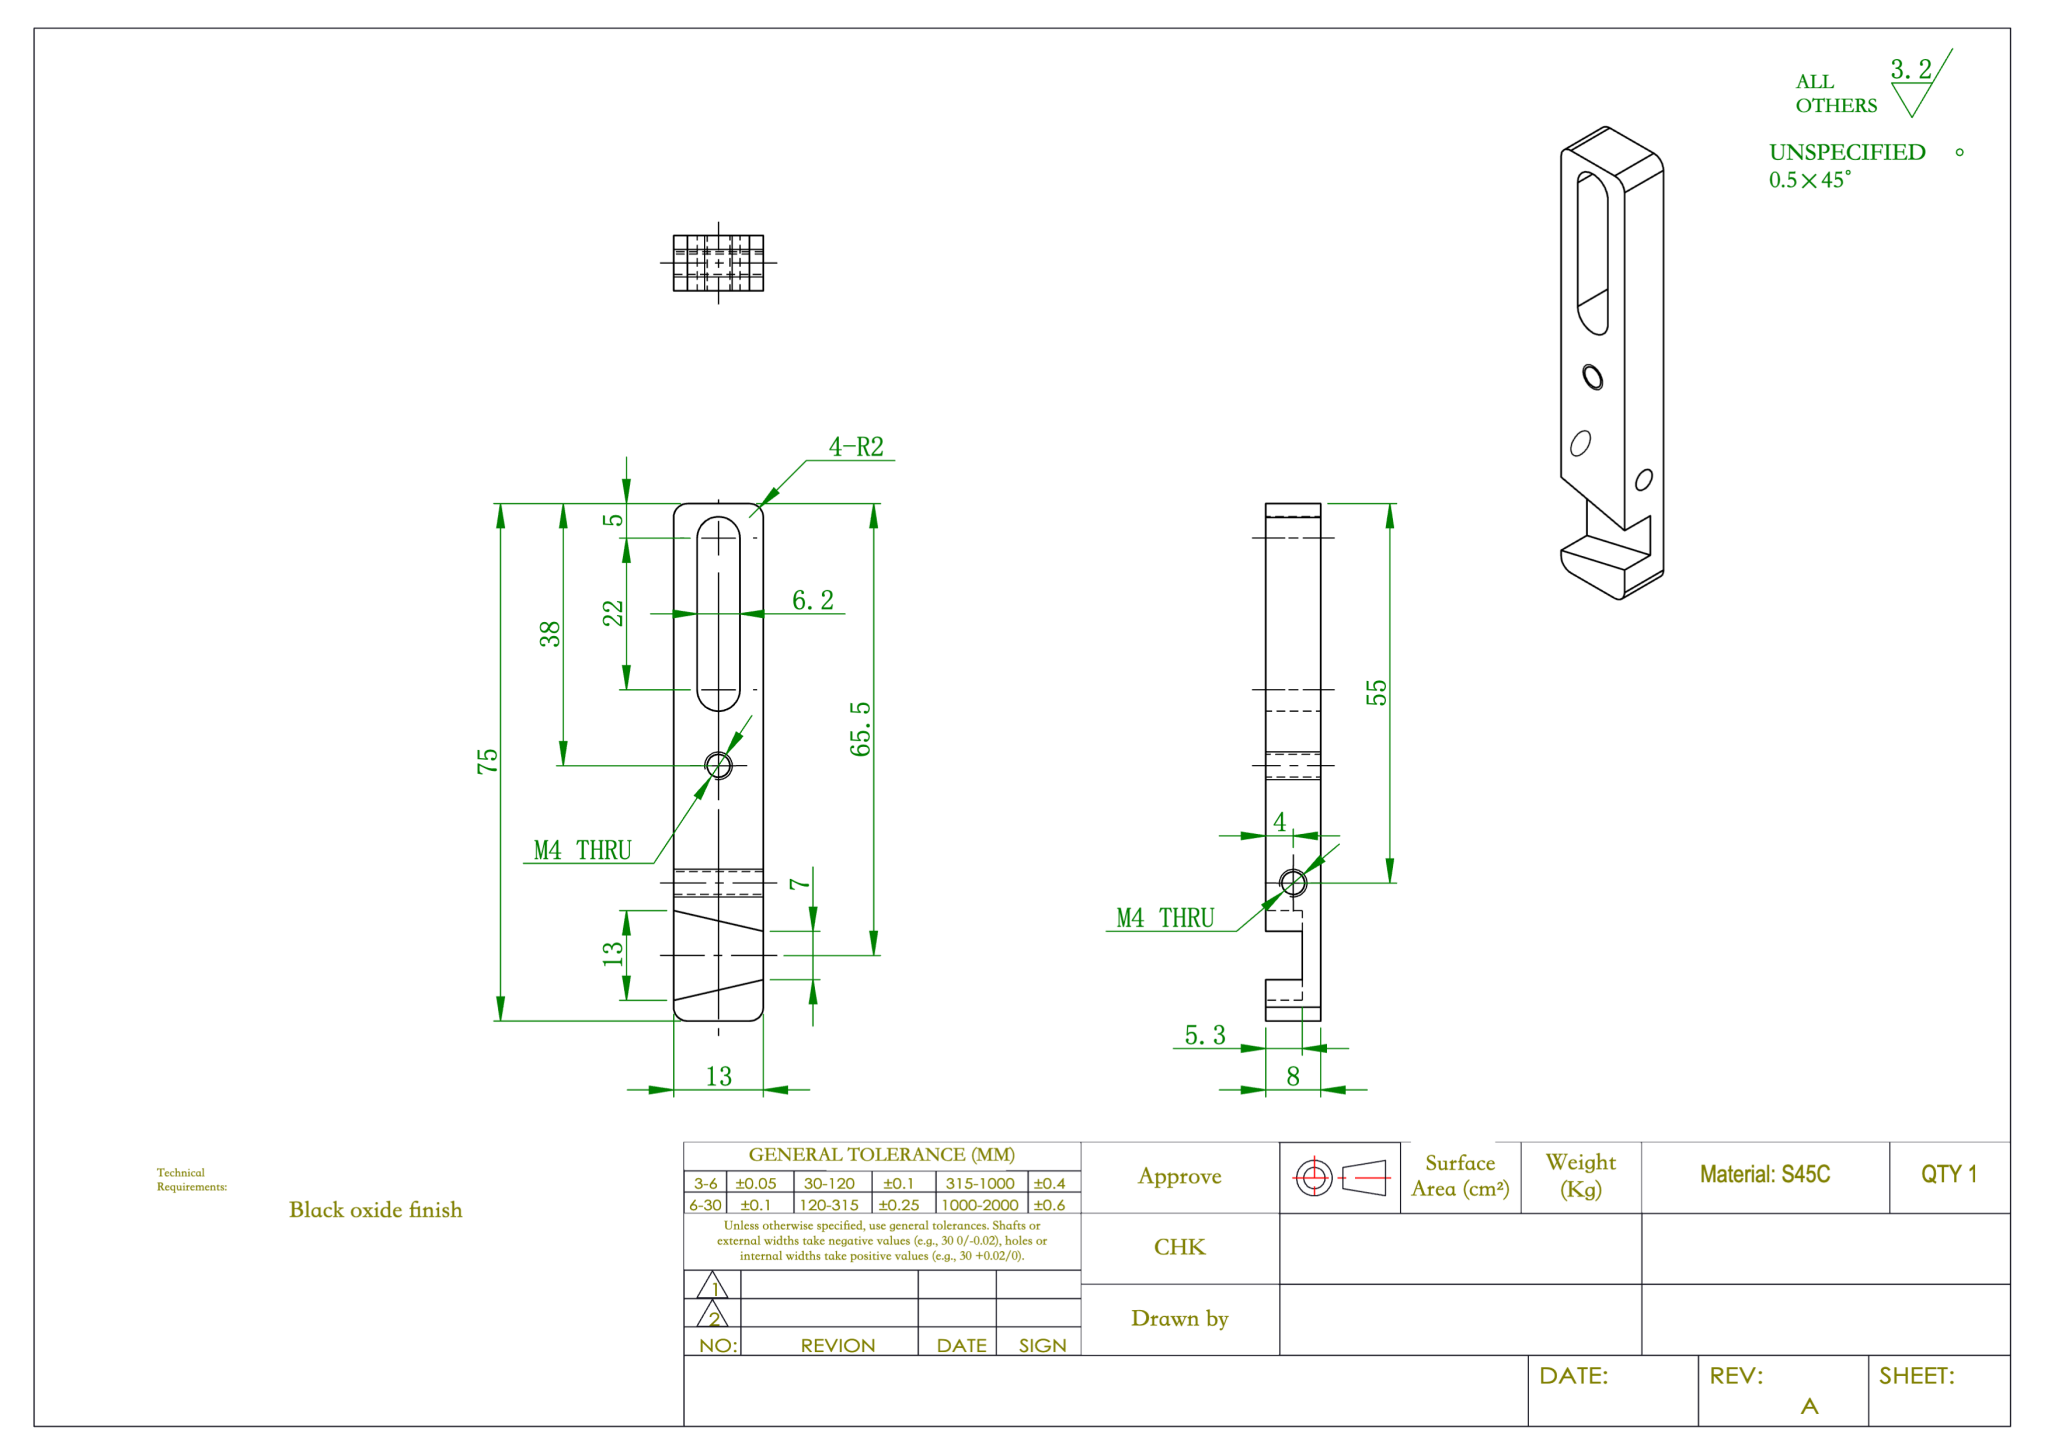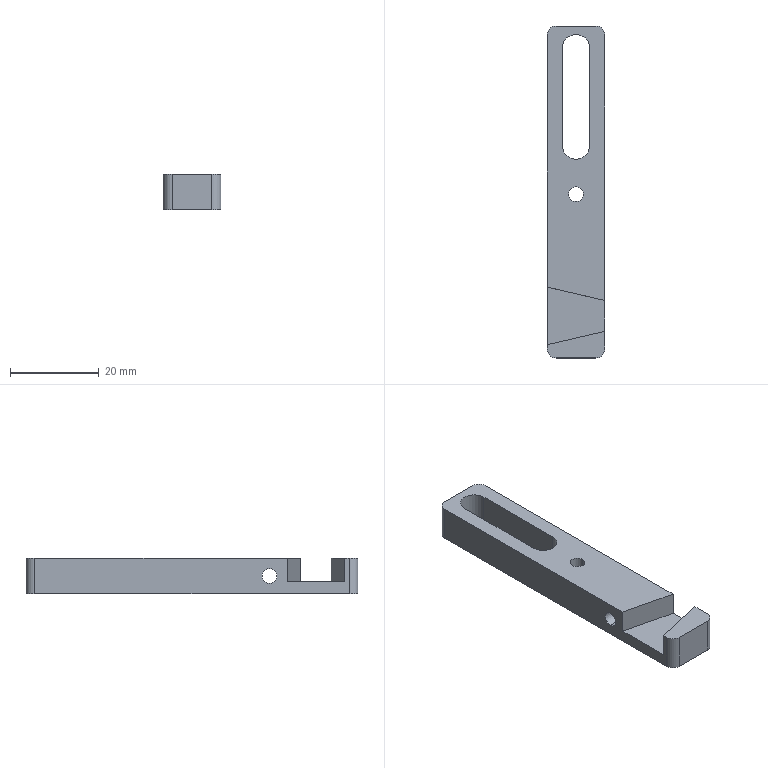Part | NX | mm | Slotted Clevis Base Bracket | 1 solid | 22 faces | box 13 x 75 x 8 mm | volume 5571 mm3 | plane 12 | cylinder 10 | commonest cylinder face diameters 3.3 x4 4 x4 6.2 x2